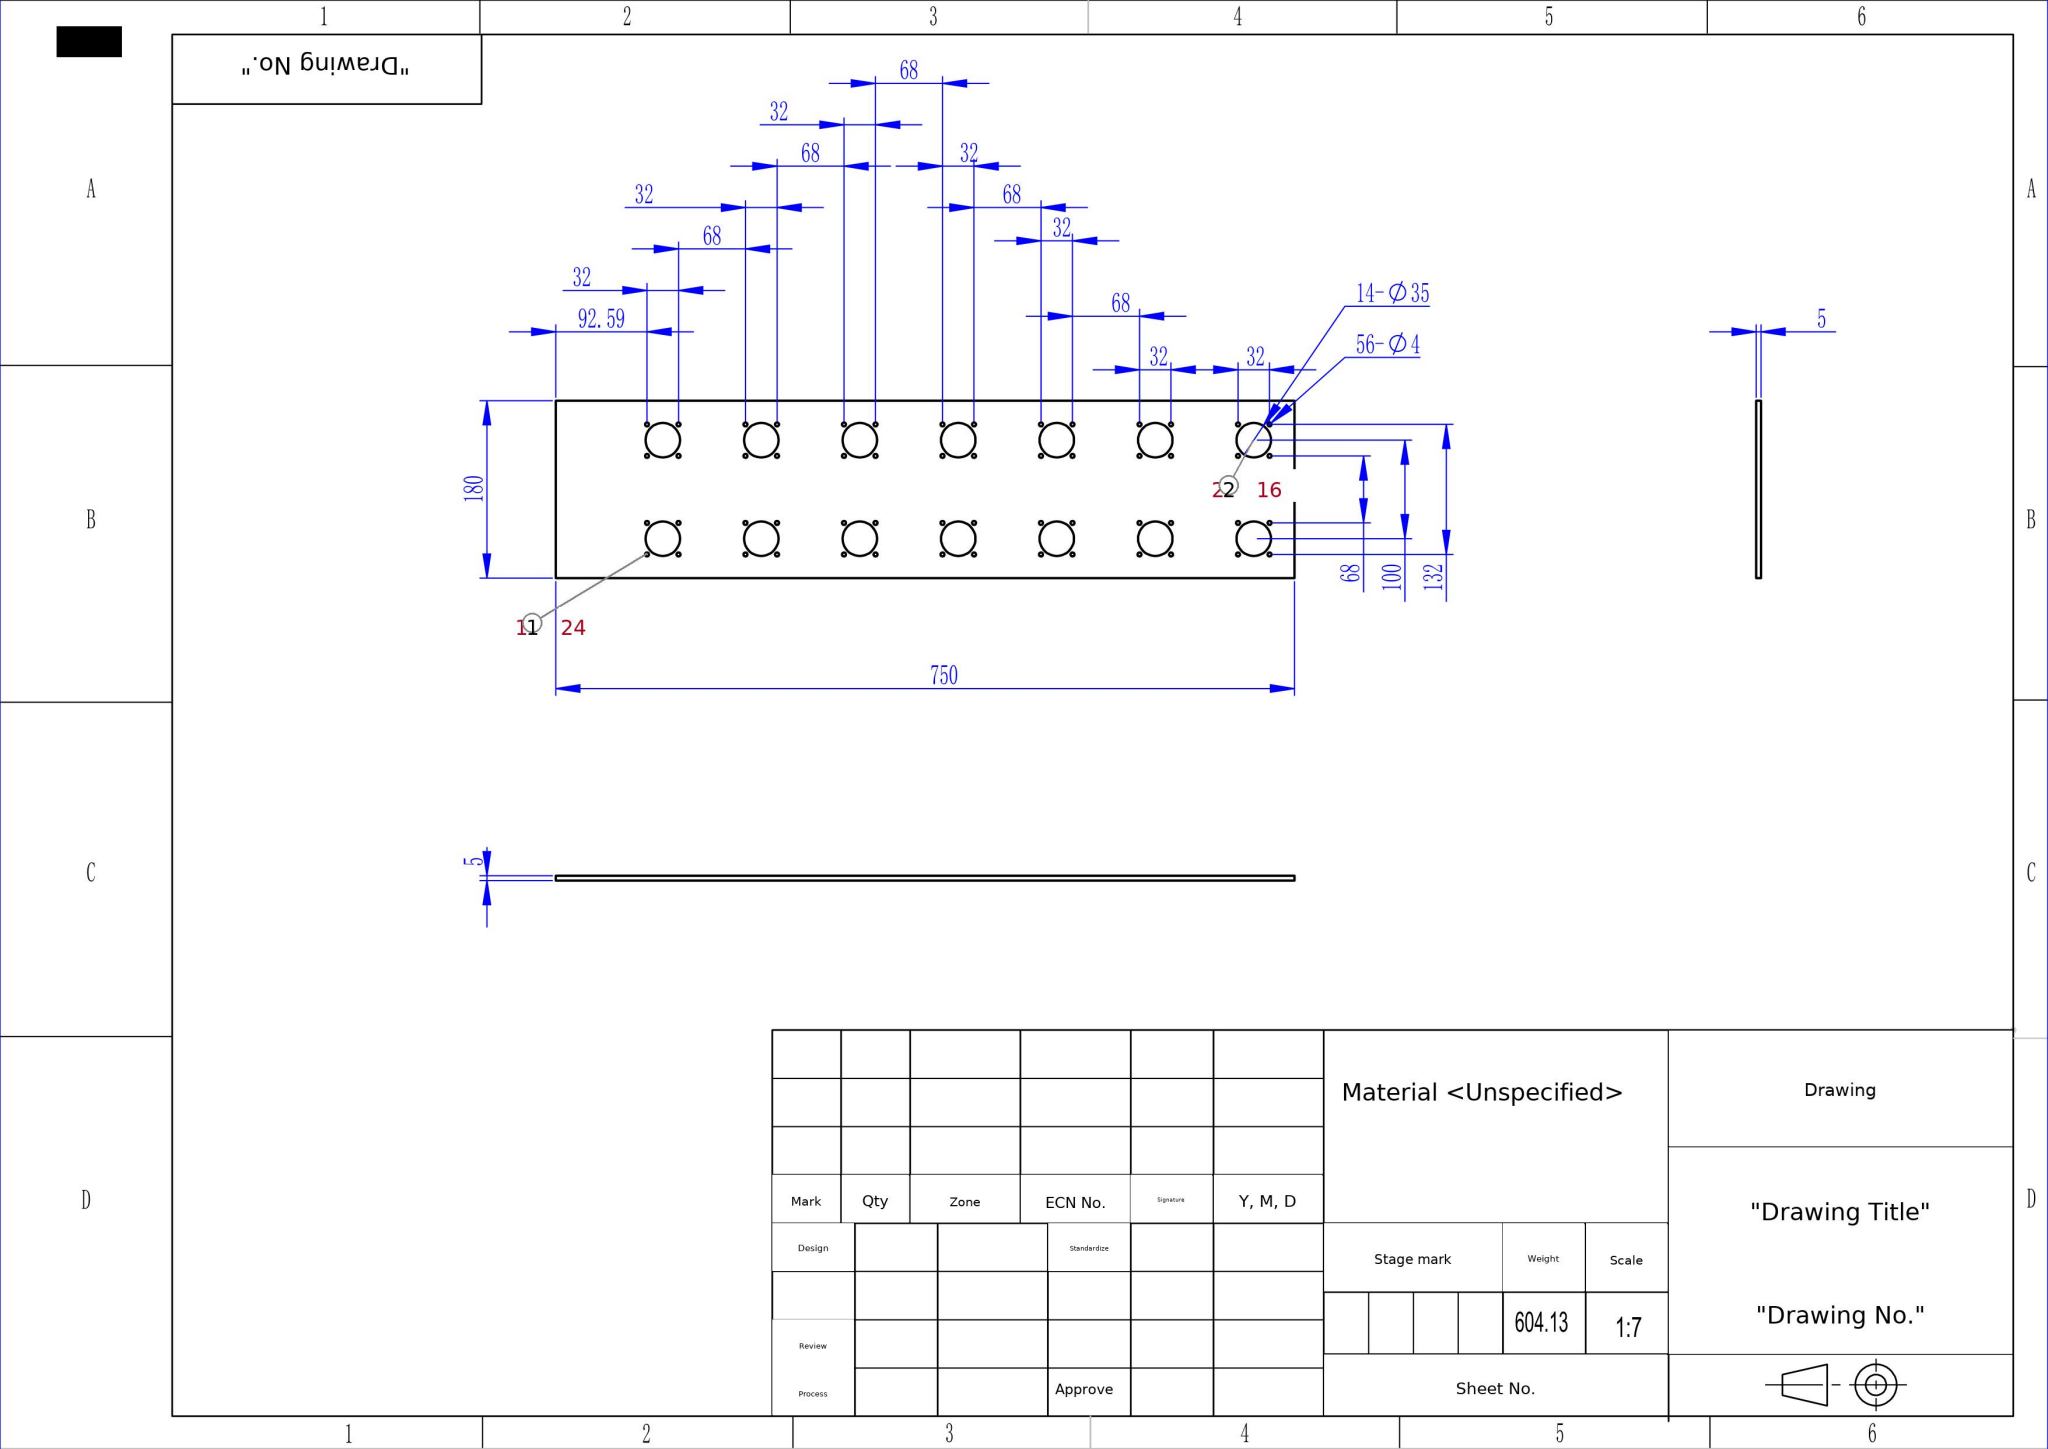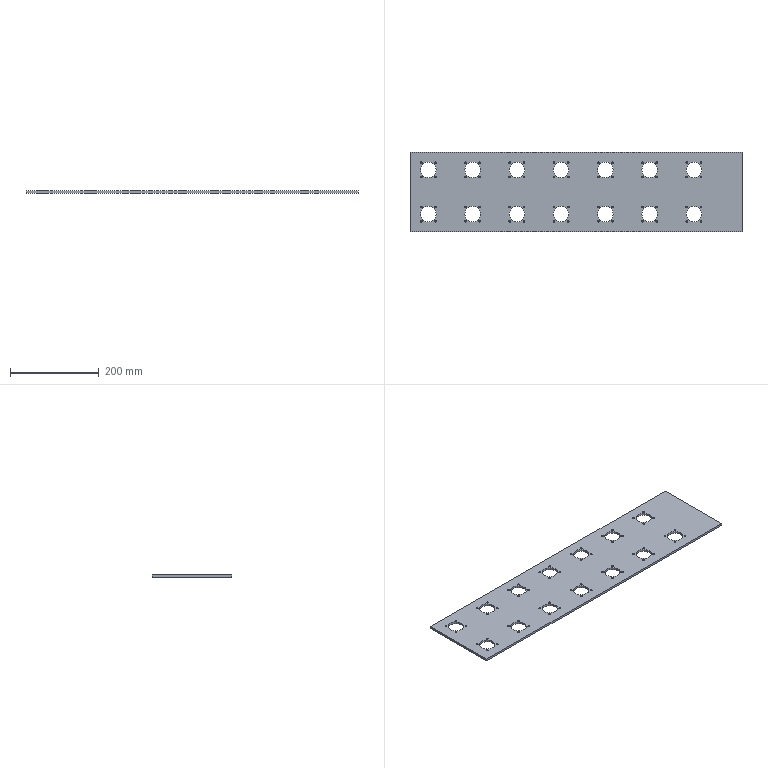Part | SolidWorks | mm | 1 solid | 146 faces | box 750 x 180 x 5 mm | volume 604134 mm3 | cylinder 140 | plane 6 | commonest cylinder face diameters 4 x112 35 x28
build123d program:
from build123d import *

# Parameters (mm, degrees)
SKETCH1_W           = 750
SKETCH1_H           = 180
SKETCH1_R           = 2
SKETCH1_R_2         = 17.5
BOSS_EXTRUDE1_DEPTH = 5


with BuildPart() as part:
    # Sketch1 → Boss-Extrude1 (new body)
    with BuildSketch(Plane.XY):
        Rectangle(SKETCH1_W, SKETCH1_H)
        with Locations((-349.585, 66)):
            Circle(SKETCH1_R, mode=Mode.SUBTRACT)
        with Locations((-317.585, 66)):
            Circle(SKETCH1_R, mode=Mode.SUBTRACT)
        with Locations((-317.585, 34)):
            Circle(SKETCH1_R, mode=Mode.SUBTRACT)
        with Locations((-349.585, 34)):
            Circle(SKETCH1_R, mode=Mode.SUBTRACT)
        with Locations((-333.585, 50)):
            Circle(SKETCH1_R_2, mode=Mode.SUBTRACT)
        with Locations((-249.585, 66)):
            Circle(SKETCH1_R, mode=Mode.SUBTRACT)
        with Locations((-217.585, 66)):
            Circle(SKETCH1_R, mode=Mode.SUBTRACT)
        with Locations((-217.585, 34)):
            Circle(SKETCH1_R, mode=Mode.SUBTRACT)
        with Locations((-249.585, 34)):
            Circle(SKETCH1_R, mode=Mode.SUBTRACT)
        with Locations((-233.585, 50)):
            Circle(SKETCH1_R_2, mode=Mode.SUBTRACT)
        with Locations((-149.585, 66)):
            Circle(SKETCH1_R, mode=Mode.SUBTRACT)
        with Locations((-117.585, 66)):
            Circle(SKETCH1_R, mode=Mode.SUBTRACT)
        with Locations((-117.585, 34)):
            Circle(SKETCH1_R, mode=Mode.SUBTRACT)
        with Locations((-149.585, 34)):
            Circle(SKETCH1_R, mode=Mode.SUBTRACT)
        with Locations((-133.585, 50)):
            Circle(SKETCH1_R_2, mode=Mode.SUBTRACT)
        with Locations((-49.585, 66)):
            Circle(SKETCH1_R, mode=Mode.SUBTRACT)
        with Locations((-17.585, 66)):
            Circle(SKETCH1_R, mode=Mode.SUBTRACT)
        with Locations((-17.585, 34)):
            Circle(SKETCH1_R, mode=Mode.SUBTRACT)
        with Locations((-49.585, 34)):
            Circle(SKETCH1_R, mode=Mode.SUBTRACT)
        with Locations((-33.585, 50)):
            Circle(SKETCH1_R_2, mode=Mode.SUBTRACT)
        with Locations((50.415, 66)):
            Circle(SKETCH1_R, mode=Mode.SUBTRACT)
        with Locations((82.415, 66)):
            Circle(SKETCH1_R, mode=Mode.SUBTRACT)
        with Locations((82.415, 34)):
            Circle(SKETCH1_R, mode=Mode.SUBTRACT)
        with Locations((50.415, 34)):
            Circle(SKETCH1_R, mode=Mode.SUBTRACT)
        with Locations((66.415, 50)):
            Circle(SKETCH1_R_2, mode=Mode.SUBTRACT)
        with Locations((150.415, 66)):
            Circle(SKETCH1_R, mode=Mode.SUBTRACT)
        with Locations((182.415, 66)):
            Circle(SKETCH1_R, mode=Mode.SUBTRACT)
        with Locations((182.415, 34)):
            Circle(SKETCH1_R, mode=Mode.SUBTRACT)
        with Locations((150.415, 34)):
            Circle(SKETCH1_R, mode=Mode.SUBTRACT)
        with Locations((166.415, 50)):
            Circle(SKETCH1_R_2, mode=Mode.SUBTRACT)
        with Locations((250.415, 66)):
            Circle(SKETCH1_R, mode=Mode.SUBTRACT)
        with Locations((282.415, 66)):
            Circle(SKETCH1_R, mode=Mode.SUBTRACT)
        with Locations((282.415, 34)):
            Circle(SKETCH1_R, mode=Mode.SUBTRACT)
        with Locations((250.415, 34)):
            Circle(SKETCH1_R, mode=Mode.SUBTRACT)
        with Locations((266.415, 50)):
            Circle(SKETCH1_R_2, mode=Mode.SUBTRACT)
        with Locations(Location((266.415, -50, 0), (0, 0, 180))):
            Circle(SKETCH1_R_2, mode=Mode.SUBTRACT)
        with Locations(Location((250.415, -34, 0), (0, 0, 180))):
            Circle(SKETCH1_R, mode=Mode.SUBTRACT)
        with Locations(Location((282.415, -34, 0), (0, 0, 180))):
            Circle(SKETCH1_R, mode=Mode.SUBTRACT)
        with Locations(Location((282.415, -66, 0), (0, 0, 180))):
            Circle(SKETCH1_R, mode=Mode.SUBTRACT)
        with Locations(Location((250.415, -66, 0), (0, 0, 180))):
            Circle(SKETCH1_R, mode=Mode.SUBTRACT)
        with Locations(Location((166.415, -50, 0), (0, 0, 180))):
            Circle(SKETCH1_R_2, mode=Mode.SUBTRACT)
        with Locations(Location((150.415, -34, 0), (0, 0, 180))):
            Circle(SKETCH1_R, mode=Mode.SUBTRACT)
        with Locations(Location((182.415, -34, 0), (0, 0, 180))):
            Circle(SKETCH1_R, mode=Mode.SUBTRACT)
        with Locations(Location((182.415, -66, 0), (0, 0, 180))):
            Circle(SKETCH1_R, mode=Mode.SUBTRACT)
        with Locations(Location((150.415, -66, 0), (0, 0, 180))):
            Circle(SKETCH1_R, mode=Mode.SUBTRACT)
        with Locations(Location((66.415, -50, 0), (0, 0, 180))):
            Circle(SKETCH1_R_2, mode=Mode.SUBTRACT)
        with Locations(Location((50.415, -34, 0), (0, 0, 180))):
            Circle(SKETCH1_R, mode=Mode.SUBTRACT)
        with Locations(Location((82.415, -34, 0), (0, 0, 180))):
            Circle(SKETCH1_R, mode=Mode.SUBTRACT)
        with Locations(Location((82.415, -66, 0), (0, 0, 180))):
            Circle(SKETCH1_R, mode=Mode.SUBTRACT)
        with Locations(Location((50.415, -66, 0), (0, 0, 180))):
            Circle(SKETCH1_R, mode=Mode.SUBTRACT)
        with Locations(Location((-33.585, -50, 0), (0, 0, 180))):
            Circle(SKETCH1_R_2, mode=Mode.SUBTRACT)
        with Locations(Location((-49.585, -34, 0), (0, 0, 180))):
            Circle(SKETCH1_R, mode=Mode.SUBTRACT)
        with Locations(Location((-17.585, -34, 0), (0, 0, 180))):
            Circle(SKETCH1_R, mode=Mode.SUBTRACT)
        with Locations(Location((-17.585, -66, 0), (0, 0, 180))):
            Circle(SKETCH1_R, mode=Mode.SUBTRACT)
        with Locations(Location((-49.585, -66, 0), (0, 0, 180))):
            Circle(SKETCH1_R, mode=Mode.SUBTRACT)
        with Locations(Location((-133.585, -50, 0), (0, 0, 180))):
            Circle(SKETCH1_R_2, mode=Mode.SUBTRACT)
        with Locations(Location((-149.585, -34, 0), (0, 0, 180))):
            Circle(SKETCH1_R, mode=Mode.SUBTRACT)
        with Locations(Location((-117.585, -34, 0), (0, 0, 180))):
            Circle(SKETCH1_R, mode=Mode.SUBTRACT)
        with Locations(Location((-117.585, -66, 0), (0, 0, 180))):
            Circle(SKETCH1_R, mode=Mode.SUBTRACT)
        with Locations(Location((-149.585, -66, 0), (0, 0, 180))):
            Circle(SKETCH1_R, mode=Mode.SUBTRACT)
        with Locations(Location((-233.585, -50, 0), (0, 0, 180))):
            Circle(SKETCH1_R_2, mode=Mode.SUBTRACT)
        with Locations(Location((-249.585, -34, 0), (0, 0, 180))):
            Circle(SKETCH1_R, mode=Mode.SUBTRACT)
        with Locations(Location((-217.585, -34, 0), (0, 0, 180))):
            Circle(SKETCH1_R, mode=Mode.SUBTRACT)
        with Locations(Location((-217.585, -66, 0), (0, 0, 180))):
            Circle(SKETCH1_R, mode=Mode.SUBTRACT)
        with Locations(Location((-249.585, -66, 0), (0, 0, 180))):
            Circle(SKETCH1_R, mode=Mode.SUBTRACT)
        with Locations(Location((-333.585, -50, 0), (0, 0, 180))):
            Circle(SKETCH1_R_2, mode=Mode.SUBTRACT)
        with Locations(Location((-349.585, -34, 0), (0, 0, 180))):
            Circle(SKETCH1_R, mode=Mode.SUBTRACT)
        with Locations(Location((-317.585, -34, 0), (0, 0, 180))):
            Circle(SKETCH1_R, mode=Mode.SUBTRACT)
        with Locations(Location((-317.585, -66, 0), (0, 0, 180))):
            Circle(SKETCH1_R, mode=Mode.SUBTRACT)
        with Locations(Location((-349.585, -66, 0), (0, 0, 180))):
            Circle(SKETCH1_R, mode=Mode.SUBTRACT)
    extrude(amount=BOSS_EXTRUDE1_DEPTH)


solid = part.part